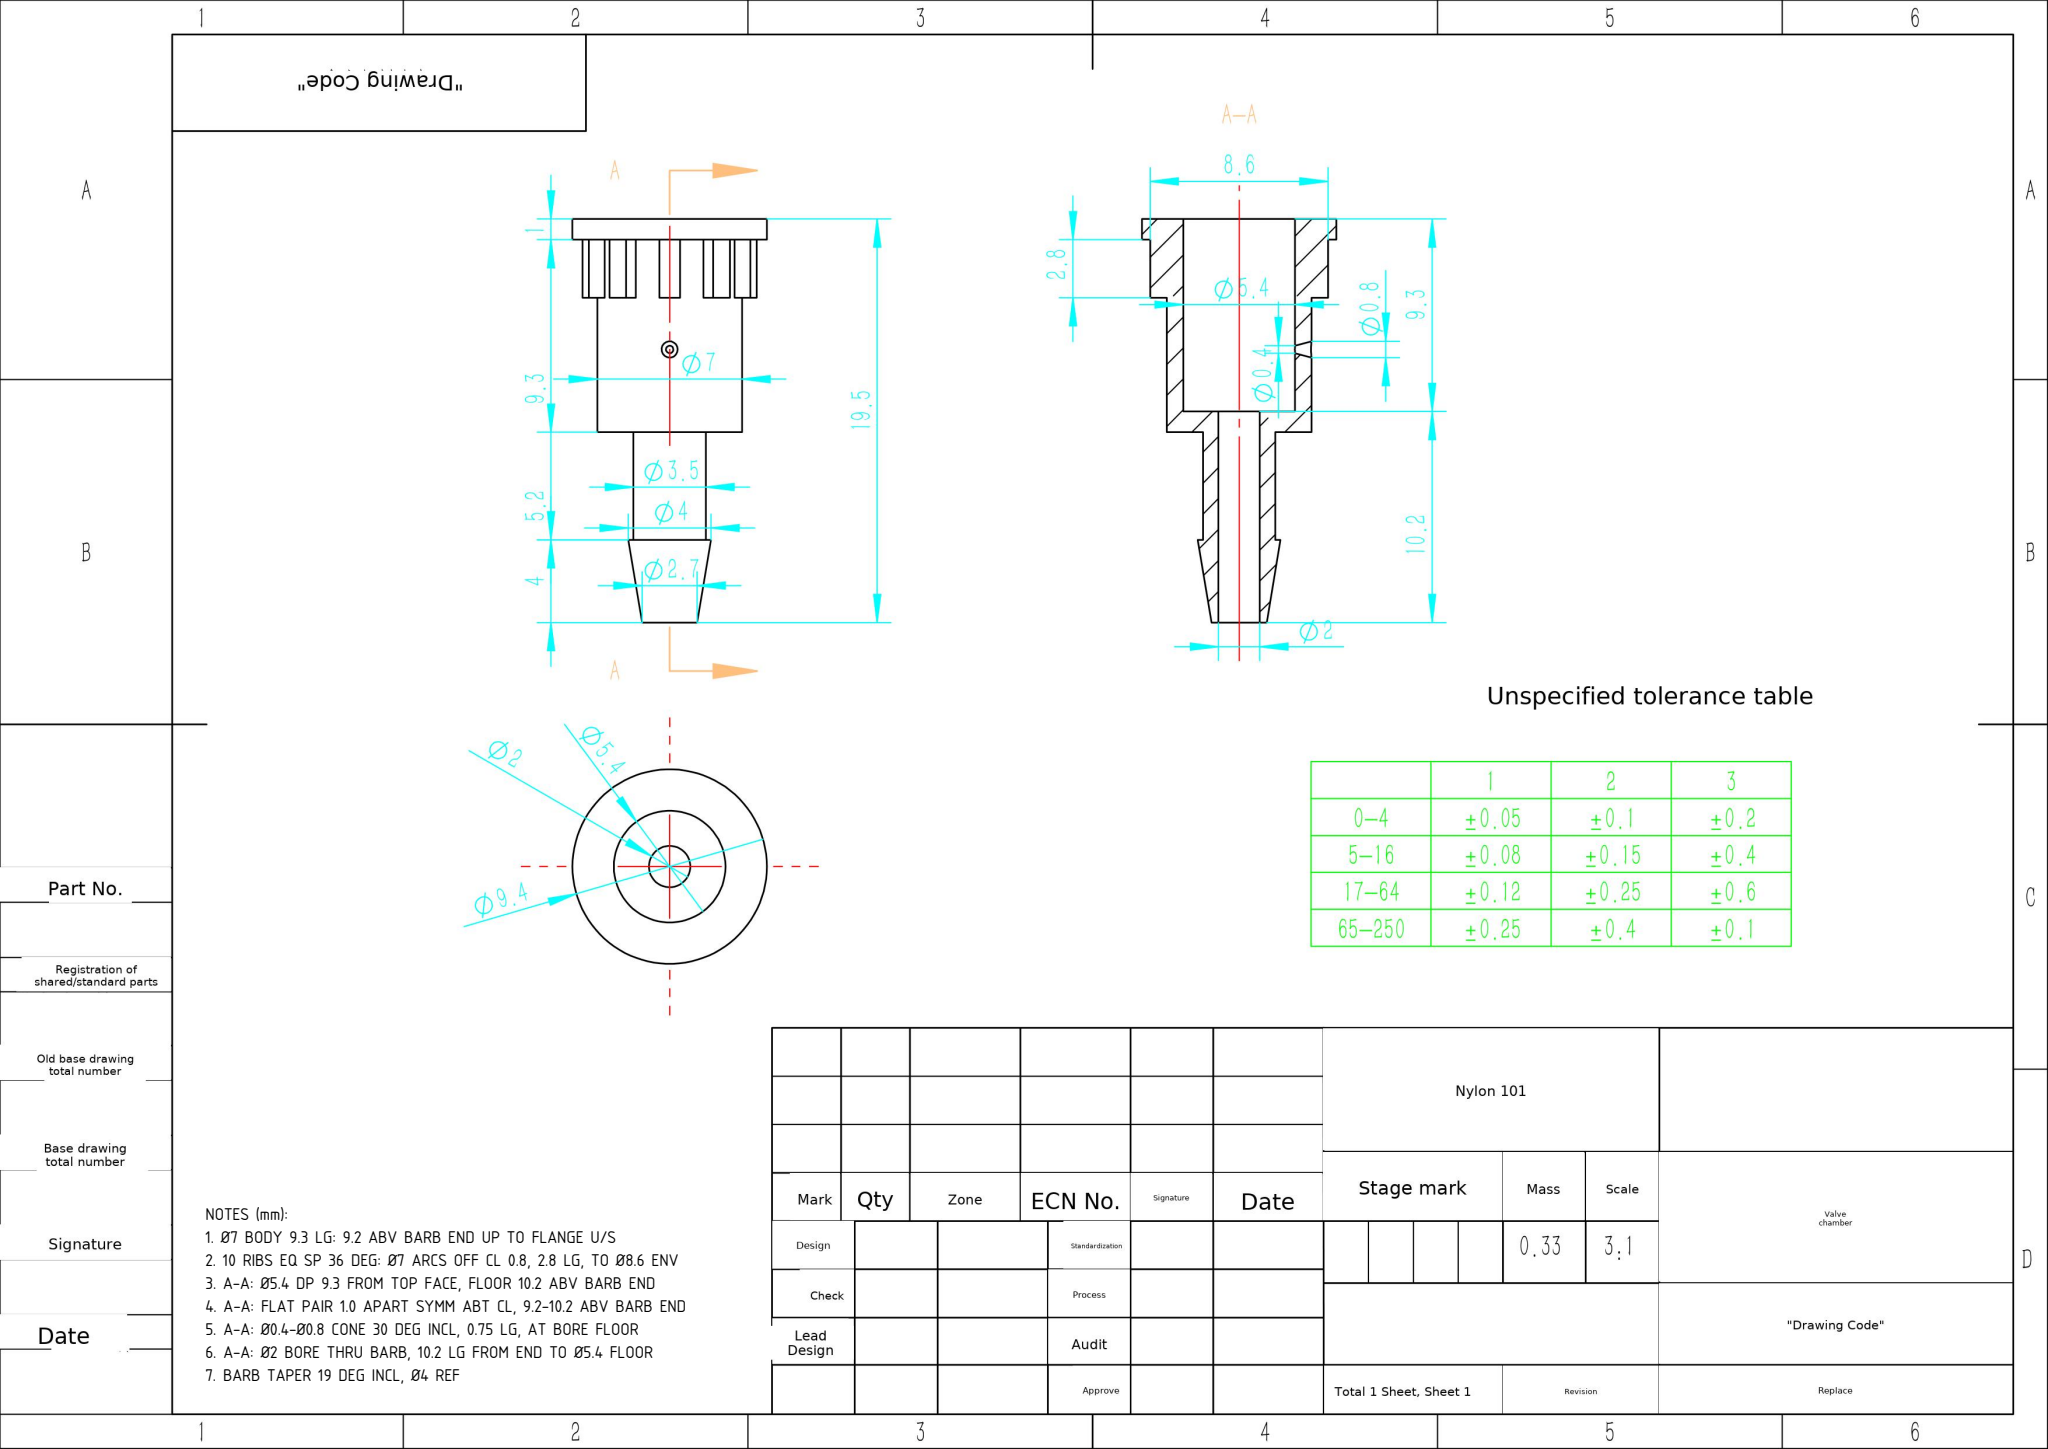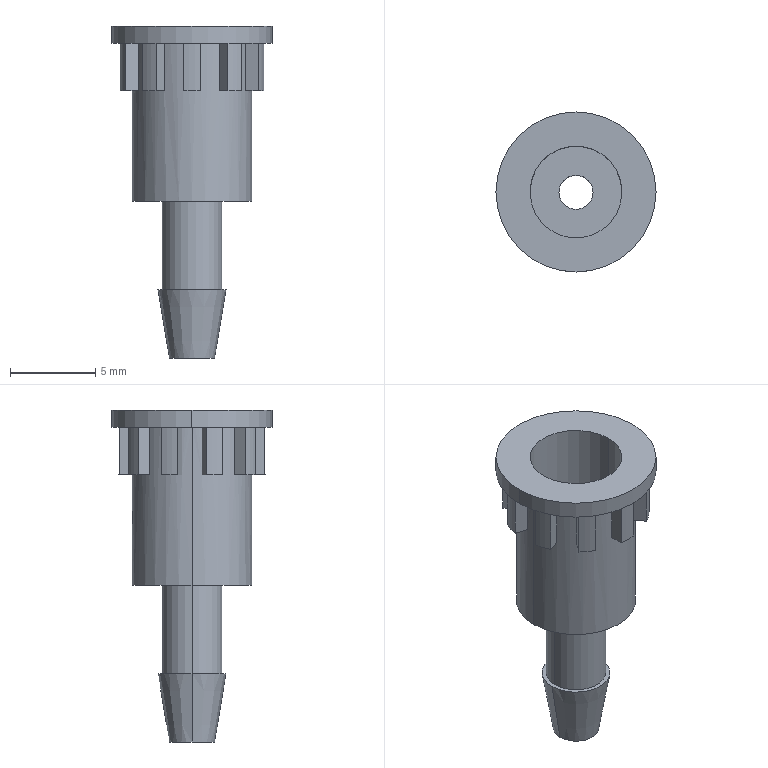Part | SolidWorks | mm | 1 solid | 60 faces | box 9.4 x 9.4 x 19.5 mm | volume 290 mm3 | plane 36 | cylinder 20 | cone 4 | commonest cylinder face diameters 7 x12 9.4 x2 3.5 x2 2 x2 5.4 x2
Drawing notes:
Ø7 BODY 9.3 LG: 9.2 ABV BARB END UP TO FLANGE U/S | from the solid: Ø7 z-cyl L=9.3 from z=9.2 to 18.5; planes z=9.2, z=18.5; bbox h=19.5
10 RIBS EQ SP 36 DEG: Ø7 ARCS OFF CL 0.8, 2.8 LG, TO Ø8.6 ENV | from the solid: 10x Ø7 z-cyl L=2.8 at r=0.8 from axis (4.7,4.7), 36° apart, z 15.7-18.5; env Ø8.6
A-A: Ø5.4 DP 9.3 FROM TOP FACE, FLOOR 10.2 ABV BARB END | from the solid: Ø5.4 z-cyl L=9.3 from z=10.2 to 19.5 top; plane z=10.2 = bore floor
A-A: FLAT PAIR 1.0 APART SYMM ABT CL, 9.2-10.2 ABV BARB END | from the solid: axis planes normal x at 4.2 and 5.2 (axis x=4.7, ±0.5); z planes 9.2 and 10.2
A-A: Ø0.4-Ø0.8 CONE 30 DEG INCL, 0.75 LG, AT BORE FLOOR | from the solid: cones[30.0,0.2]: Ø0.4 small end -> Ø0.8; axial lg=(0.8-0.4)/2/tan15°=0.75; floor z=10.2
A-A: Ø2 BORE THRU BARB, 10.2 LG FROM END TO Ø5.4 FLOOR | from the solid: Ø2 z-cyl L=10.2 from z=0 to 10.2
BARB TAPER 19 DEG INCL, Ø4 REF | from the solid: cones[19.0,4.0] x2 at barb end
build123d program:
from build123d import *

# Parameters (mm, degrees)
SKETCH1_R                  = 1.75
BOSS_EXTRUDE1_DEPTH        = 5.2
SKETCH2_R                  = 2
BOSS_EXTRUDE2_DEPTH        = 4
BOSS_EXTRUDE2_TAPER        = 9.5
SKETCH3_R                  = 3.5
BOSS_EXTRUDE3_DEPTH        = 10.3
BOSS_EXTRUDE4_REACH        = 19.071
BOSS_EXTRUDE4_START_RADIUS = 3.5
BOSS_EXTRUDE4_END_RADIUS   = 3.5
SKETCH4_W                  = 1
SKETCH4_H                  = 3.8
CIRPATTERN1_COUNT          = 10
SKETCH5_R                  = 1
CUT_EXTRUDE1_DEPTH         = 21.407
SKETCH6_R                  = 2.7
CUT_EXTRUDE2_DEPTH         = 9.3
CUT_EXTRUDE3_START         = 2.4
SKETCH7_R                  = 0.1
CUT_EXTRUDE3_DEPTH         = 15.227
CUT_EXTRUDE3_DRAFT         = -15
SKETCH8_R                  = 4.7
SKETCH8_R_2                = 2.7
BOSS_EXTRUDE5_DEPTH        = 1


with BuildPart() as part:
    # Sketch1 → Boss-Extrude1 (new body)
    with BuildSketch(Plane.XY):
        Circle(SKETCH1_R)
    extrude(amount=BOSS_EXTRUDE1_DEPTH)

    # Sketch2 → Boss-Extrude2 (add)
    with BuildSketch(Plane(origin=(0, 0, 0), x_dir=(-1, 0, 0), z_dir=(0, 0, -1))):
        Circle(SKETCH2_R)
    extrude(amount=BOSS_EXTRUDE2_DEPTH, taper=BOSS_EXTRUDE2_TAPER)

    # Sketch3 → Boss-Extrude3 (add)
    with BuildSketch(Plane.XY.offset(5.2)):
        with Locations(Location((0, 0, 0), (0, 0, 180))):
            Circle(SKETCH3_R)
    extrude(amount=BOSS_EXTRUDE3_DEPTH)

    # Boss-Extrude4: from a cylinder face, 19.071 long prism both ways, kept between that surface and its translate by the depth
    boss_extrude4_start = Plane(origin=(0, 0, 13.6), z_dir=(0, 0, -1)) * Cylinder(BOSS_EXTRUDE4_START_RADIUS, 46.142, mode=Mode.PRIVATE)
    boss_extrude4_end = Plane(origin=(0, 0.8, 13.6), z_dir=(0, 0, -1)) * Cylinder(BOSS_EXTRUDE4_END_RADIUS, 46.142, mode=Mode.PRIVATE)
    # Sketch4 → Boss-Extrude4 (add, from a surface)
    with BuildSketch(Plane(origin=(0, 0, 0), x_dir=(1, 0, 0), z_dir=(0, 1, 0)), mode=Mode.PRIVATE) as boss_extrude4_sk1:
        with Locations((0, -13.6)):
            Rectangle(SKETCH4_W, SKETCH4_H)
    boss_extrude4_tool1 = extrude(boss_extrude4_sk1.sketch, amount=BOSS_EXTRUDE4_REACH, both=True, mode=Mode.PRIVATE)
    boss_extrude4 = ((boss_extrude4_tool1 - boss_extrude4_start) & boss_extrude4_end).solids().sort_by_distance((0, 3.864, 13.6))[0]
    add(boss_extrude4)

    # CirPattern1: Boss-Extrude4 ×10 about axis
    cirpattern1_axis = Axis((0, 0, 0), (0, 0, 1))
    for i in range(1, CIRPATTERN1_COUNT):
        add(boss_extrude4.rotate(cirpattern1_axis, i * 360 / CIRPATTERN1_COUNT))

    # Sketch5 → Cut-Extrude1 (cut, through all)
    with BuildSketch(Plane(origin=(0, 0, -4), x_dir=(-1, 0, 0), z_dir=(0, 0, -1))):
        Circle(SKETCH5_R)
    extrude(amount=-CUT_EXTRUDE1_DEPTH, mode=Mode.SUBTRACT)

    # Sketch6 → Cut-Extrude2 (cut)
    with BuildSketch(Plane.XY.offset(15.5)):
        Circle(SKETCH6_R)
    extrude(amount=-CUT_EXTRUDE2_DEPTH, mode=Mode.SUBTRACT)


with BuildPart() as cut_extrude3_tool:
    # Sketch7 → Cut-Extrude3 (with draft: the straight prism first)
    with BuildSketch(Plane(origin=(0, 0, 0), x_dir=(1, 0, 0), z_dir=(0, 1, 0)).offset(CUT_EXTRUDE3_START)):
        with Locations((0, -9.2)):
            Circle(SKETCH7_R)
    extrude(amount=CUT_EXTRUDE3_DEPTH)
    # Cut-Extrude3: the draft: its side faces are tilted about the plane it starts from
    cut_extrude3_sides = [cut_extrude3_tool.faces().sort_by_distance(p)[0] for p in [
        (-0.1, 10.014, 9.2),
    ]]
    draft(cut_extrude3_sides, Plane(origin=(0, 0, 0), x_dir=(1, 0, 0), z_dir=(0, 1, 0)).offset(CUT_EXTRUDE3_START), CUT_EXTRUDE3_DRAFT)


with BuildPart() as part_1:
    add(part.part)

    # Cut-Extrude3: cut by cut_extrude3_tool
    add(cut_extrude3_tool.part, mode=Mode.SUBTRACT)

    # Sketch8 → Boss-Extrude5 (add)
    with BuildSketch(Plane.XY.offset(15.5)):
        Circle(SKETCH8_R)
        Circle(SKETCH8_R_2, mode=Mode.SUBTRACT)
    extrude(amount=-BOSS_EXTRUDE5_DEPTH)


solid = part_1.part